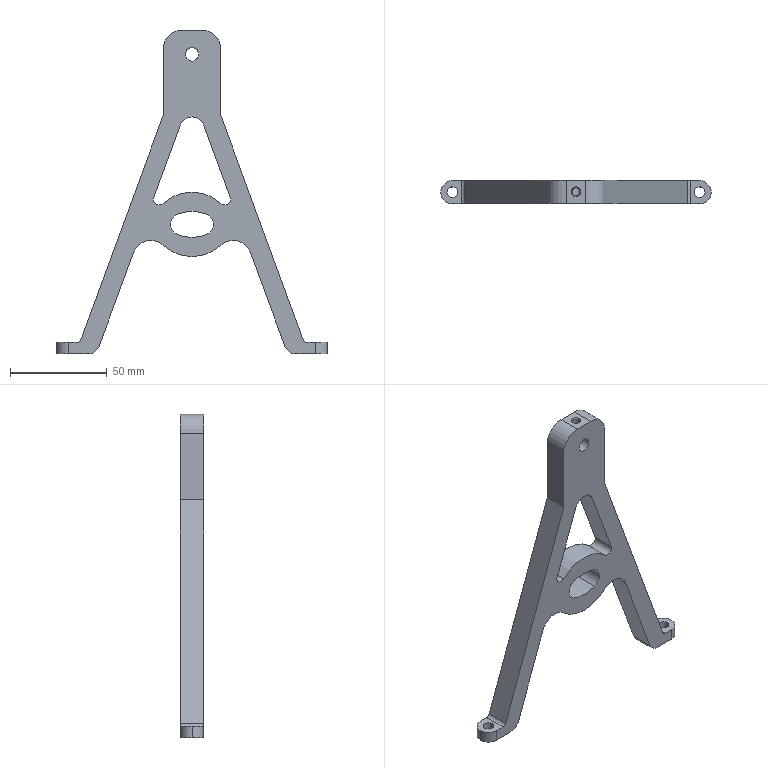Component | NX | BRACKET | 1 solid | 41 faces | volume 59999 mm3 | cylinder 25 | plane 15 | cone 1 | commonest cylinder face diameters 12 x6 4 x3 20 x2 11.32 x2 40.003 x2 5.946 x2 44 x2 18.853 x2